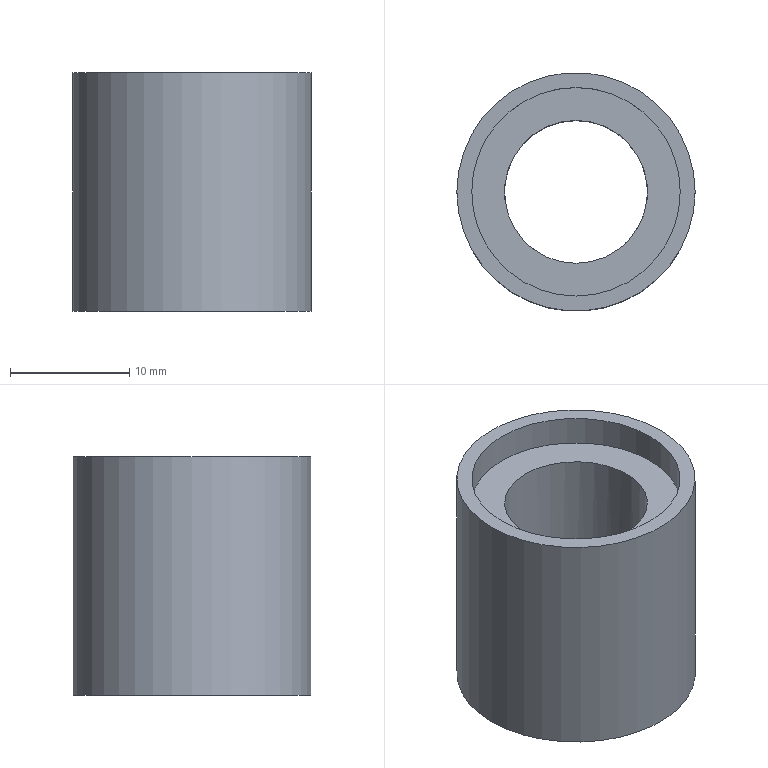Component | NX | LINER_BUSH | 1 solid | 6 faces | box 20 x 20 x 20 mm | volume 3703 mm3 | cylinder 3 | plane 3 | commonest cylinder face diameters 20 x1 12 x1 17.5 x1
STEP:
#1=CARTESIAN_POINT('',(0.,0.,0.));
#2=DIRECTION('',(0.,0.,1.));
#3=DIRECTION('',(1.,0.,0.));
#4=AXIS2_PLACEMENT_3D('',#1,#2,#3);
#5=CARTESIAN_POINT('',(10.,-1.,148.));
#6=VERTEX_POINT('',#5);
#7=CARTESIAN_POINT('',(0.,-1.,148.));
#8=DIRECTION('',(0.,0.,-1.));
#9=DIRECTION('',(1.,0.,0.));
#10=AXIS2_PLACEMENT_3D('',#7,#8,#9);
#11=CIRCLE('',#10,10.);
#12=CARTESIAN_POINT('',(0.,-1.,148.));
#13=DIRECTION('',(0.,0.,-1.));
#14=DIRECTION('',(0.,1.,0.));
#15=AXIS2_PLACEMENT_3D('',#12,#13,#14);
#16=CYLINDRICAL_SURFACE('',#15,10.);
#17=CARTESIAN_POINT('',(1.571,0.));
#18=DIRECTION('',(1.,0.));
#19=VECTOR('',#18,1.);
#20=LINE('',#17,#19);
#21=(GEOMETRIC_REPRESENTATION_CONTEXT(2)PARAMETRIC_REPRESENTATION_CONTEXT()REPRESENTATION_CONTEXT('',''));
#22=DEFINITIONAL_REPRESENTATION('',(#20),#21);
#23=PCURVE('',#16,#22);
#24=CARTESIAN_POINT('',(0.,-1.,148.));
#25=DIRECTION('',(0.,0.,-1.));
#26=DIRECTION('',(0.,1.,0.));
#27=AXIS2_PLACEMENT_3D('',#24,#25,#26);
#28=PLANE('',#27);
#29=CARTESIAN_POINT('',(0.,0.));
#30=DIRECTION('',(0.,1.));
#31=AXIS2_PLACEMENT_2D('',#29,#30);
#32=CIRCLE('',#31,10.);
#33=(GEOMETRIC_REPRESENTATION_CONTEXT(2)PARAMETRIC_REPRESENTATION_CONTEXT()REPRESENTATION_CONTEXT('',''));
#34=DEFINITIONAL_REPRESENTATION('',(#32),#33);
#35=PCURVE('',#28,#34);
#36=SURFACE_CURVE('',#11,(#23,#35),.PCURVE_S1.);
#37=EDGE_CURVE('',#6,#6,#36,.T.);
#38=ORIENTED_EDGE('',*,*,#37,.T.);
#39=CARTESIAN_POINT('',(10.,-1.,128.));
#40=VERTEX_POINT('',#39);
#41=CARTESIAN_POINT('',(10.,-1.,148.));
#42=CARTESIAN_POINT('',(10.,-1.,128.));
#43=B_SPLINE_CURVE_WITH_KNOTS('',1,(#41,#42),.UNSPECIFIED.,.F.,.F.,(2,2),(0.,20.),.PIECEWISE_BEZIER_KNOTS.);
#44=CARTESIAN_POINT('',(7.854,0.));
#45=DIRECTION('',(0.,1.));
#46=VECTOR('',#45,1.);
#47=LINE('',#44,#46);
#48=(GEOMETRIC_REPRESENTATION_CONTEXT(2)PARAMETRIC_REPRESENTATION_CONTEXT()REPRESENTATION_CONTEXT('',''));
#49=DEFINITIONAL_REPRESENTATION('',(#47),#48);
#50=PCURVE('',#16,#49);
#51=CARTESIAN_POINT('',(1.571,0.));
#52=DIRECTION('',(0.,1.));
#53=VECTOR('',#52,1.);
#54=LINE('',#51,#53);
#55=(GEOMETRIC_REPRESENTATION_CONTEXT(2)PARAMETRIC_REPRESENTATION_CONTEXT()REPRESENTATION_CONTEXT('',''));
#56=DEFINITIONAL_REPRESENTATION('',(#54),#55);
#57=PCURVE('',#16,#56);
#58=SEAM_CURVE('',#43,(#50,#57),.PCURVE_S1.);
#59=EDGE_CURVE('',#6,#40,#58,.T.);
#60=ORIENTED_EDGE('',*,*,#59,.T.);
#61=CARTESIAN_POINT('',(0.,-1.,128.));
#62=DIRECTION('',(0.,0.,-1.));
#63=DIRECTION('',(1.,0.,0.));
#64=AXIS2_PLACEMENT_3D('',#61,#62,#63);
#65=CIRCLE('',#64,10.);
#66=CARTESIAN_POINT('',(1.571,20.));
#67=DIRECTION('',(1.,0.));
#68=VECTOR('',#67,1.);
#69=LINE('',#66,#68);
#70=(GEOMETRIC_REPRESENTATION_CONTEXT(2)PARAMETRIC_REPRESENTATION_CONTEXT()REPRESENTATION_CONTEXT('',''));
#71=DEFINITIONAL_REPRESENTATION('',(#69),#70);
#72=PCURVE('',#16,#71);
#73=CARTESIAN_POINT('',(0.,-1.,128.));
#74=DIRECTION('',(0.,0.,-1.));
#75=DIRECTION('',(0.,1.,0.));
#76=AXIS2_PLACEMENT_3D('',#73,#74,#75);
#77=PLANE('',#76);
#78=CARTESIAN_POINT('',(0.,0.));
#79=DIRECTION('',(0.,1.));
#80=AXIS2_PLACEMENT_2D('',#78,#79);
#81=CIRCLE('',#80,10.);
#82=(GEOMETRIC_REPRESENTATION_CONTEXT(2)PARAMETRIC_REPRESENTATION_CONTEXT()REPRESENTATION_CONTEXT('',''));
#83=DEFINITIONAL_REPRESENTATION('',(#81),#82);
#84=PCURVE('',#77,#83);
#85=SURFACE_CURVE('',#65,(#72,#84),.PCURVE_S1.);
#86=EDGE_CURVE('',#40,#40,#85,.T.);
#87=ORIENTED_EDGE('',*,*,#86,.F.);
#88=ORIENTED_EDGE('',*,*,#59,.F.);
#89=EDGE_LOOP('',(#38,#60,#87,#88));
#90=FACE_BOUND('',#89,.T.);
#91=ADVANCED_FACE('',(#90),#16,.T.);
#92=CARTESIAN_POINT('',(0.,5.,145.5));
#93=VERTEX_POINT('',#92);
#94=CARTESIAN_POINT('',(0.,-1.,145.5));
#95=DIRECTION('',(0.,0.,1.));
#96=DIRECTION('',(0.,1.,0.));
#97=AXIS2_PLACEMENT_3D('',#94,#95,#96);
#98=CIRCLE('',#97,6.);
#99=CARTESIAN_POINT('',(0.,-1.,148.));
#100=DIRECTION('',(0.,0.,-1.));
#101=DIRECTION('',(0.,1.,0.));
#102=AXIS2_PLACEMENT_3D('',#99,#100,#101);
#103=CYLINDRICAL_SURFACE('',#102,6.);
#104=CARTESIAN_POINT('',(6.283,2.5));
#105=DIRECTION('',(-1.,0.));
#106=VECTOR('',#105,1.);
#107=LINE('',#104,#106);
#108=(GEOMETRIC_REPRESENTATION_CONTEXT(2)PARAMETRIC_REPRESENTATION_CONTEXT()REPRESENTATION_CONTEXT('',''));
#109=DEFINITIONAL_REPRESENTATION('',(#107),#108);
#110=PCURVE('',#103,#109);
#111=CARTESIAN_POINT('',(0.,-1.,145.5));
#112=DIRECTION('',(0.,0.,-1.));
#113=DIRECTION('',(0.,1.,0.));
#114=AXIS2_PLACEMENT_3D('',#111,#112,#113);
#115=PLANE('',#114);
#116=CARTESIAN_POINT('',(6.,0.));
#117=CARTESIAN_POINT('',(6.,-10.392));
#118=CARTESIAN_POINT('',(-3.,-5.196));
#119=CARTESIAN_POINT('',(-12.,-0.));
#120=CARTESIAN_POINT('',(-3.,5.196));
#121=CARTESIAN_POINT('',(6.,10.392));
#122=CARTESIAN_POINT('',(6.,0.));
#123=(BOUNDED_CURVE()B_SPLINE_CURVE(2,(#116,#117,#118,#119,#120,#121,#122),.UNSPECIFIED.,.T.,.F.)B_SPLINE_CURVE_WITH_KNOTS((1,2,2,2,2,1),(-2.094,0.,2.094,4.189,6.283,8.378),.UNSPECIFIED.)CURVE()GEOMETRIC_REPRESENTATION_ITEM()RATIONAL_B_SPLINE_CURVE((1.,0.5,1.,0.5,1.,0.5,1.))REPRESENTATION_ITEM(''));
#124=(GEOMETRIC_REPRESENTATION_CONTEXT(2)PARAMETRIC_REPRESENTATION_CONTEXT()REPRESENTATION_CONTEXT('',''));
#125=DEFINITIONAL_REPRESENTATION('',(#123),#124);
#126=PCURVE('',#115,#125);
#127=SURFACE_CURVE('',#98,(#110,#126),.PCURVE_S1.);
#128=EDGE_CURVE('',#93,#93,#127,.T.);
#129=ORIENTED_EDGE('',*,*,#128,.F.);
#130=CARTESIAN_POINT('',(-0.,5.,128.));
#131=VERTEX_POINT('',#130);
#132=CARTESIAN_POINT('',(0.,5.,145.5));
#133=CARTESIAN_POINT('',(0.,5.,128.));
#134=B_SPLINE_CURVE_WITH_KNOTS('',1,(#132,#133),.UNSPECIFIED.,.F.,.F.,(2,2),(2.5,20.),.PIECEWISE_BEZIER_KNOTS.);
#135=CARTESIAN_POINT('',(6.283,0.));
#136=DIRECTION('',(0.,1.));
#137=VECTOR('',#136,1.);
#138=LINE('',#135,#137);
#139=(GEOMETRIC_REPRESENTATION_CONTEXT(2)PARAMETRIC_REPRESENTATION_CONTEXT()REPRESENTATION_CONTEXT('',''));
#140=DEFINITIONAL_REPRESENTATION('',(#138),#139);
#141=PCURVE('',#103,#140);
#142=CARTESIAN_POINT('',(0.,0.));
#143=DIRECTION('',(0.,1.));
#144=VECTOR('',#143,1.);
#145=LINE('',#142,#144);
#146=(GEOMETRIC_REPRESENTATION_CONTEXT(2)PARAMETRIC_REPRESENTATION_CONTEXT()REPRESENTATION_CONTEXT('',''));
#147=DEFINITIONAL_REPRESENTATION('',(#145),#146);
#148=PCURVE('',#103,#147);
#149=SEAM_CURVE('',#134,(#141,#148),.PCURVE_S1.);
#150=EDGE_CURVE('',#93,#131,#149,.T.);
#151=ORIENTED_EDGE('',*,*,#150,.T.);
#152=CARTESIAN_POINT('',(6.,-1.,128.));
#153=VERTEX_POINT('',#152);
#154=CARTESIAN_POINT('',(0.,-1.,128.));
#155=DIRECTION('',(0.,0.,-1.));
#156=DIRECTION('',(1.,0.,0.));
#157=AXIS2_PLACEMENT_3D('',#154,#155,#156);
#158=CIRCLE('',#157,6.);
#159=CARTESIAN_POINT('',(1.571,20.));
#160=DIRECTION('',(1.,0.));
#161=VECTOR('',#160,1.);
#162=LINE('',#159,#161);
#163=(GEOMETRIC_REPRESENTATION_CONTEXT(2)PARAMETRIC_REPRESENTATION_CONTEXT()REPRESENTATION_CONTEXT('',''));
#164=DEFINITIONAL_REPRESENTATION('',(#162),#163);
#165=PCURVE('',#103,#164);
#166=CARTESIAN_POINT('',(0.,0.));
#167=DIRECTION('',(0.,1.));
#168=AXIS2_PLACEMENT_2D('',#166,#167);
#169=CIRCLE('',#168,6.);
#170=(GEOMETRIC_REPRESENTATION_CONTEXT(2)PARAMETRIC_REPRESENTATION_CONTEXT()REPRESENTATION_CONTEXT('',''));
#171=DEFINITIONAL_REPRESENTATION('',(#169),#170);
#172=PCURVE('',#77,#171);
#173=SURFACE_CURVE('',#158,(#165,#172),.PCURVE_S1.);
#174=EDGE_CURVE('',#153,#131,#173,.T.);
#175=ORIENTED_EDGE('',*,*,#174,.F.);
#176=CARTESIAN_POINT('',(0.,-1.,128.));
#177=DIRECTION('',(0.,0.,-1.));
#178=DIRECTION('',(1.,0.,0.));
#179=AXIS2_PLACEMENT_3D('',#176,#177,#178);
#180=CIRCLE('',#179,6.);
#181=CARTESIAN_POINT('',(-4.712,20.));
#182=DIRECTION('',(1.,0.));
#183=VECTOR('',#182,1.);
#184=LINE('',#181,#183);
#185=(GEOMETRIC_REPRESENTATION_CONTEXT(2)PARAMETRIC_REPRESENTATION_CONTEXT()REPRESENTATION_CONTEXT('',''));
#186=DEFINITIONAL_REPRESENTATION('',(#184),#185);
#187=PCURVE('',#103,#186);
#188=CARTESIAN_POINT('',(0.,0.));
#189=DIRECTION('',(0.,1.));
#190=AXIS2_PLACEMENT_2D('',#188,#189);
#191=CIRCLE('',#190,6.);
#192=(GEOMETRIC_REPRESENTATION_CONTEXT(2)PARAMETRIC_REPRESENTATION_CONTEXT()REPRESENTATION_CONTEXT('',''));
#193=DEFINITIONAL_REPRESENTATION('',(#191),#192);
#194=PCURVE('',#77,#193);
#195=SURFACE_CURVE('',#180,(#187,#194),.PCURVE_S1.);
#196=EDGE_CURVE('',#131,#153,#195,.T.);
#197=ORIENTED_EDGE('',*,*,#196,.F.);
#198=ORIENTED_EDGE('',*,*,#150,.F.);
#199=EDGE_LOOP('',(#129,#151,#175,#197,#198));
#200=FACE_BOUND('',#199,.F.);
#201=ADVANCED_FACE('',(#200),#103,.F.);
#202=CARTESIAN_POINT('',(0.,7.75,148.));
#203=VERTEX_POINT('',#202);
#204=CARTESIAN_POINT('',(8.75,-1.,148.));
#205=VERTEX_POINT('',#204);
#206=CARTESIAN_POINT('',(0.,-1.,148.));
#207=DIRECTION('',(0.,0.,-1.));
#208=DIRECTION('',(0.,1.,0.));
#209=AXIS2_PLACEMENT_3D('',#206,#207,#208);
#210=CIRCLE('',#209,8.75);
#211=CARTESIAN_POINT('',(0.,0.));
#212=DIRECTION('',(1.,0.));
#213=AXIS2_PLACEMENT_2D('',#211,#212);
#214=CIRCLE('',#213,8.75);
#215=(GEOMETRIC_REPRESENTATION_CONTEXT(2)PARAMETRIC_REPRESENTATION_CONTEXT()REPRESENTATION_CONTEXT('',''));
#216=DEFINITIONAL_REPRESENTATION('',(#214),#215);
#217=PCURVE('',#28,#216);
#218=CARTESIAN_POINT('',(0.,-1.,145.5));
#219=DIRECTION('',(0.,0.,1.));
#220=DIRECTION('',(1.,0.,0.));
#221=AXIS2_PLACEMENT_3D('',#218,#219,#220);
#222=CYLINDRICAL_SURFACE('',#221,8.75);
#223=CARTESIAN_POINT('',(1.571,2.5));
#224=DIRECTION('',(-1.,0.));
#225=VECTOR('',#224,1.);
#226=LINE('',#223,#225);
#227=(GEOMETRIC_REPRESENTATION_CONTEXT(2)PARAMETRIC_REPRESENTATION_CONTEXT()REPRESENTATION_CONTEXT('',''));
#228=DEFINITIONAL_REPRESENTATION('',(#226),#227);
#229=PCURVE('',#222,#228);
#230=SURFACE_CURVE('',#210,(#217,#229),.PCURVE_S1.);
#231=EDGE_CURVE('',#203,#205,#230,.T.);
#232=ORIENTED_EDGE('',*,*,#231,.T.);
#233=CARTESIAN_POINT('',(0.,-1.,148.));
#234=DIRECTION('',(0.,0.,-1.));
#235=DIRECTION('',(0.,1.,0.));
#236=AXIS2_PLACEMENT_3D('',#233,#234,#235);
#237=CIRCLE('',#236,8.75);
#238=CARTESIAN_POINT('',(0.,0.));
#239=DIRECTION('',(1.,0.));
#240=AXIS2_PLACEMENT_2D('',#238,#239);
#241=CIRCLE('',#240,8.75);
#242=(GEOMETRIC_REPRESENTATION_CONTEXT(2)PARAMETRIC_REPRESENTATION_CONTEXT()REPRESENTATION_CONTEXT('',''));
#243=DEFINITIONAL_REPRESENTATION('',(#241),#242);
#244=PCURVE('',#28,#243);
#245=CARTESIAN_POINT('',(7.854,2.5));
#246=DIRECTION('',(-1.,0.));
#247=VECTOR('',#246,1.);
#248=LINE('',#245,#247);
#249=(GEOMETRIC_REPRESENTATION_CONTEXT(2)PARAMETRIC_REPRESENTATION_CONTEXT()REPRESENTATION_CONTEXT('',''));
#250=DEFINITIONAL_REPRESENTATION('',(#248),#249);
#251=PCURVE('',#222,#250);
#252=SURFACE_CURVE('',#237,(#244,#251),.PCURVE_S1.);
#253=EDGE_CURVE('',#205,#203,#252,.T.);
#254=ORIENTED_EDGE('',*,*,#253,.T.);
#255=EDGE_LOOP('',(#232,#254));
#256=FACE_BOUND('',#255,.T.);
#257=ORIENTED_EDGE('',*,*,#37,.F.);
#258=EDGE_LOOP('',(#257));
#259=FACE_BOUND('',#258,.T.);
#260=ADVANCED_FACE('',(#256,#259),#28,.F.);
#261=ORIENTED_EDGE('',*,*,#86,.T.);
#262=EDGE_LOOP('',(#261));
#263=FACE_BOUND('',#262,.T.);
#264=ORIENTED_EDGE('',*,*,#174,.F.);
#265=ORIENTED_EDGE('',*,*,#196,.F.);
#266=EDGE_LOOP('',(#264,#265));
#267=FACE_BOUND('',#266,.T.);
#268=ADVANCED_FACE('',(#263,#267),#77,.T.);
#269=CARTESIAN_POINT('',(8.75,-1.,145.5));
#270=VERTEX_POINT('',#269);
#271=CARTESIAN_POINT('',(0.,-1.,145.5));
#272=DIRECTION('',(0.,0.,-1.));
#273=DIRECTION('',(1.,0.,0.));
#274=AXIS2_PLACEMENT_3D('',#271,#272,#273);
#275=CIRCLE('',#274,8.75);
#276=CARTESIAN_POINT('',(0.,0.));
#277=DIRECTION('',(0.,1.));
#278=AXIS2_PLACEMENT_2D('',#276,#277);
#279=CIRCLE('',#278,8.75);
#280=(GEOMETRIC_REPRESENTATION_CONTEXT(2)PARAMETRIC_REPRESENTATION_CONTEXT()REPRESENTATION_CONTEXT('',''));
#281=DEFINITIONAL_REPRESENTATION('',(#279),#280);
#282=PCURVE('',#115,#281);
#283=CARTESIAN_POINT('',(6.283,0.));
#284=DIRECTION('',(-1.,0.));
#285=VECTOR('',#284,1.);
#286=LINE('',#283,#285);
#287=(GEOMETRIC_REPRESENTATION_CONTEXT(2)PARAMETRIC_REPRESENTATION_CONTEXT()REPRESENTATION_CONTEXT('',''));
#288=DEFINITIONAL_REPRESENTATION('',(#286),#287);
#289=PCURVE('',#222,#288);
#290=SURFACE_CURVE('',#275,(#282,#289),.PCURVE_S1.);
#291=EDGE_CURVE('',#270,#270,#290,.T.);
#292=ORIENTED_EDGE('',*,*,#291,.F.);
#293=EDGE_LOOP('',(#292));
#294=FACE_BOUND('',#293,.T.);
#295=ORIENTED_EDGE('',*,*,#128,.F.);
#296=EDGE_LOOP('',(#295));
#297=FACE_BOUND('',#296,.T.);
#298=ADVANCED_FACE('',(#294,#297),#115,.F.);
#299=ORIENTED_EDGE('',*,*,#291,.F.);
#300=CARTESIAN_POINT('',(8.75,-1.,145.5));
#301=CARTESIAN_POINT('',(8.75,-1.,148.));
#302=B_SPLINE_CURVE_WITH_KNOTS('',1,(#300,#301),.UNSPECIFIED.,.F.,.F.,(2,2),(0.,2.5),.PIECEWISE_BEZIER_KNOTS.);
#303=CARTESIAN_POINT('',(6.283,0.));
#304=DIRECTION('',(0.,1.));
#305=VECTOR('',#304,1.);
#306=LINE('',#303,#305);
#307=(GEOMETRIC_REPRESENTATION_CONTEXT(2)PARAMETRIC_REPRESENTATION_CONTEXT()REPRESENTATION_CONTEXT('',''));
#308=DEFINITIONAL_REPRESENTATION('',(#306),#307);
#309=PCURVE('',#222,#308);
#310=CARTESIAN_POINT('',(0.,0.));
#311=DIRECTION('',(0.,1.));
#312=VECTOR('',#311,1.);
#313=LINE('',#310,#312);
#314=(GEOMETRIC_REPRESENTATION_CONTEXT(2)PARAMETRIC_REPRESENTATION_CONTEXT()REPRESENTATION_CONTEXT('',''));
#315=DEFINITIONAL_REPRESENTATION('',(#313),#314);
#316=PCURVE('',#222,#315);
#317=SEAM_CURVE('',#302,(#309,#316),.PCURVE_S1.);
#318=EDGE_CURVE('',#270,#205,#317,.T.);
#319=ORIENTED_EDGE('',*,*,#318,.T.);
#320=ORIENTED_EDGE('',*,*,#253,.T.);
#321=ORIENTED_EDGE('',*,*,#231,.T.);
#322=ORIENTED_EDGE('',*,*,#318,.F.);
#323=EDGE_LOOP('',(#299,#319,#320,#321,#322));
#324=FACE_BOUND('',#323,.F.);
#325=ADVANCED_FACE('',(#324),#222,.F.);
#326=CLOSED_SHELL('',(#91,#201,#260,#268,#298,#325));
#327=MANIFOLD_SOLID_BREP('',#326);
#328=(LENGTH_UNIT()NAMED_UNIT(*)SI_UNIT(.MILLI.,.METRE.));
#329=UNCERTAINTY_MEASURE_WITH_UNIT(LENGTH_MEASURE(0.000005),#328,'','');
#330=(NAMED_UNIT(*)PLANE_ANGLE_UNIT()SI_UNIT($,.RADIAN.));
#331=(NAMED_UNIT(*)SI_UNIT($,.STERADIAN.)SOLID_ANGLE_UNIT());
#332=(GEOMETRIC_REPRESENTATION_CONTEXT(3)GLOBAL_UNCERTAINTY_ASSIGNED_CONTEXT((#329))GLOBAL_UNIT_ASSIGNED_CONTEXT((#328,#330,#331))REPRESENTATION_CONTEXT('',''));
#333=ADVANCED_BREP_SHAPE_REPRESENTATION('',(#4,#327),#332);